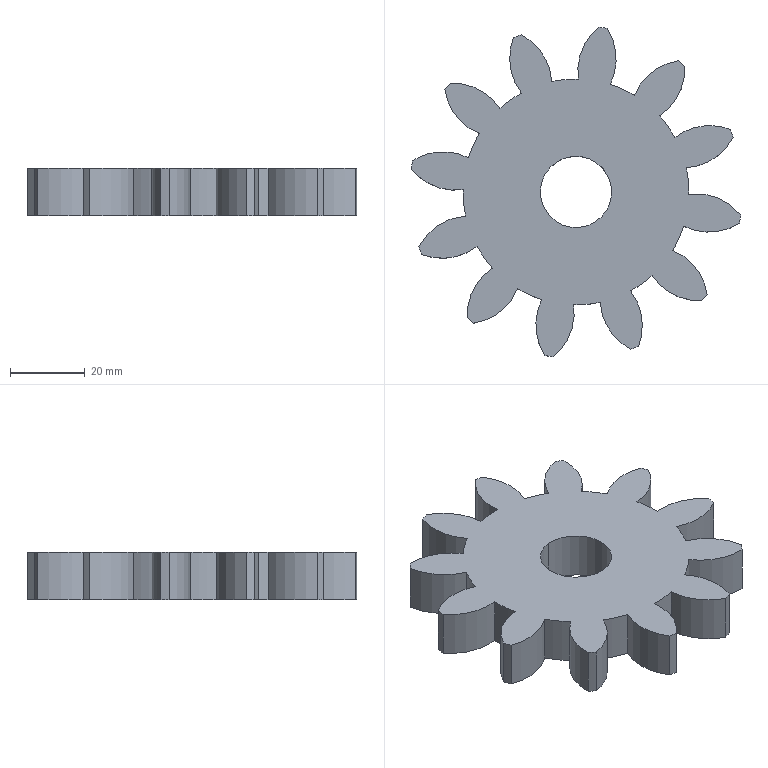Component | SolidWorks | spur gear_gb-7 | 1 solid | 57 faces | volume 50526 mm3 | cylinder 55 | plane 2 | commonest cylinder face diameters 30.48 x28 60.322 x13 88.9 x12 19.05 x2